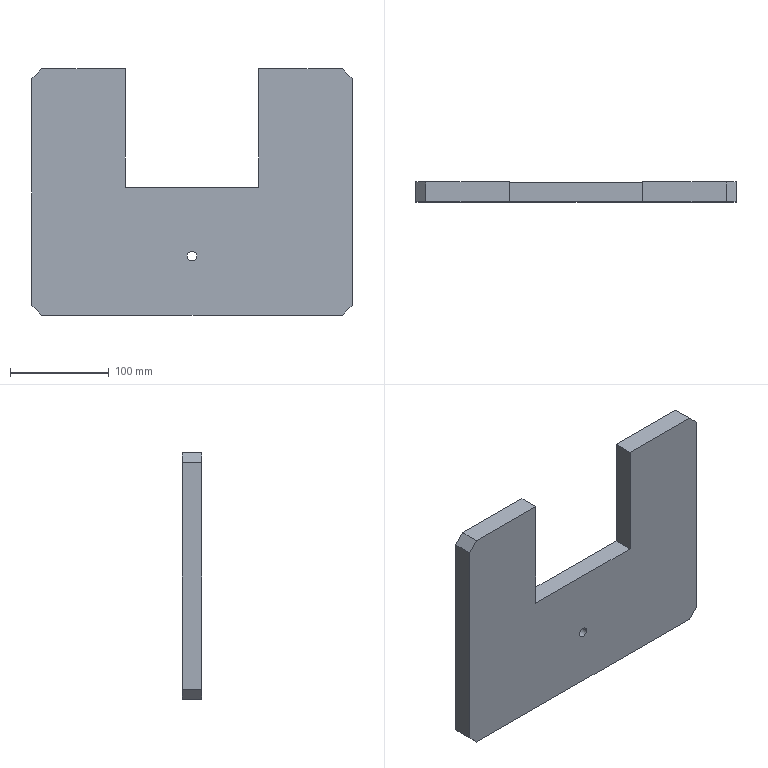Component | SolidWorks | RobotGripperBasePlateB-1 | 1 solid | 16 faces | box 325 x 20 x 250 mm | volume 1295429 mm3 | plane 14 | cylinder 2 | commonest cylinder face diameters 10 x2 | material Aviation Aluminum-7075
build123d program:
from build123d import *

# Parameters (mm, degrees)
SKETCH1_W           = 325
SKETCH1_H           = 250
BOSS_EXTRUDE1_DEPTH = 20
CHAMFER1_SIZE       = 10
SKETCH2_R           = 5
CUT_EXTRUDE1_DEPTH  = 206.988
CHAMFER2_SIZE       = 10
SKETCH3_W           = 135
SKETCH3_H           = 120
CUT_EXTRUDE2_DEPTH  = 206.988


with BuildPart() as part:
    # Sketch1 → Boss-Extrude1 (new body)
    with BuildSketch(Plane.XY):
        Rectangle(SKETCH1_W, SKETCH1_H)
    extrude(amount=BOSS_EXTRUDE1_DEPTH)

    # Chamfer1
    chamfer1_edges = [part.edges().sort_by_distance(p)[0] for p in [
        (-162.5, 125, 10),
        (162.5, 125, 10),
    ]]
    chamfer(chamfer1_edges, length=CHAMFER1_SIZE)

    # Sketch2 → Cut-Extrude1 (cut, through all)
    with BuildSketch(Plane.XY.offset(20)):
        with Locations((0, 65)):
            Circle(SKETCH2_R)
    extrude(amount=-CUT_EXTRUDE1_DEPTH, mode=Mode.SUBTRACT)

    # Chamfer2
    chamfer2_edges = [part.edges().sort_by_distance(p)[0] for p in [
        (162.5, -125, 10),
        (-162.5, -125, 10),
    ]]
    chamfer(chamfer2_edges, length=CHAMFER2_SIZE)

    # Sketch3 → Cut-Extrude2 (cut, through all)
    with BuildSketch(Plane(origin=(0, 0, 0), x_dir=(-1, 0, 0), z_dir=(0, 0, -1))):
        with Locations((0, -65)):
            Rectangle(SKETCH3_W, SKETCH3_H)
    extrude(amount=-CUT_EXTRUDE2_DEPTH, mode=Mode.SUBTRACT)


solid = part.part

# Placed as in the assembly
solid = solid.moved(Location((-47.37, -204.626, 352.215), (-90, 0, 0)))
STEP:
#1=COLOUR_RGB('',0.7922,0.8196,0.9333);
#2=FILL_AREA_STYLE_COLOUR('',#1);
#3=FILL_AREA_STYLE('',(#2));
#4=SURFACE_STYLE_FILL_AREA(#3);
#5=SURFACE_SIDE_STYLE('',(#4));
#6=SURFACE_STYLE_USAGE(.BOTH.,#5);
#7=PRESENTATION_STYLE_ASSIGNMENT((#6));
#8=CARTESIAN_POINT('',(-1.668,-7.269,11.308));
#9=VERTEX_POINT('',#8);
#10=CARTESIAN_POINT('',(-2.062,-7.269,11.308));
#11=VERTEX_POINT('',#10);
#12=CARTESIAN_POINT('',(-1.865,-7.269,11.308));
#13=DIRECTION('',(-0.,-1.,0.));
#14=DIRECTION('',(-1.,0.,0.));
#15=AXIS2_PLACEMENT_3D('',#12,#13,#14);
#16=CIRCLE('',#15,0.1969);
#17=EDGE_CURVE('',#9,#11,#16,.T.);
#18=ORIENTED_EDGE('',*,*,#17,.F.);
#19=CARTESIAN_POINT('',(-1.668,-8.056,11.308));
#20=VERTEX_POINT('',#19);
#21=CARTESIAN_POINT('',(-1.668,-7.269,11.308));
#22=DIRECTION('',(-0.,-1.,0.));
#23=VECTOR('',#22,39.37);
#24=LINE('',#21,#23);
#25=EDGE_CURVE('',#9,#20,#24,.T.);
#26=ORIENTED_EDGE('',*,*,#25,.T.);
#27=CARTESIAN_POINT('',(-2.062,-8.056,11.308));
#28=VERTEX_POINT('',#27);
#29=CARTESIAN_POINT('',(-1.865,-8.056,11.308));
#30=DIRECTION('',(-0.,-1.,0.));
#31=DIRECTION('',(-1.,0.,0.));
#32=AXIS2_PLACEMENT_3D('',#29,#30,#31);
#33=CIRCLE('',#32,0.1969);
#34=EDGE_CURVE('',#20,#28,#33,.T.);
#35=ORIENTED_EDGE('',*,*,#34,.T.);
#36=CARTESIAN_POINT('',(-2.062,-7.269,11.308));
#37=DIRECTION('',(-0.,-1.,0.));
#38=VECTOR('',#37,39.37);
#39=LINE('',#36,#38);
#40=EDGE_CURVE('',#11,#28,#39,.T.);
#41=ORIENTED_EDGE('',*,*,#40,.F.);
#42=EDGE_LOOP('',(#18,#26,#35,#41));
#43=FACE_OUTER_BOUND('',#42,.T.);
#44=CARTESIAN_POINT('',(-1.865,-7.269,11.308));
#45=DIRECTION('',(-0.,-1.,0.));
#46=DIRECTION('',(-1.,0.,0.));
#47=AXIS2_PLACEMENT_3D('',#44,#45,#46);
#48=CYLINDRICAL_SURFACE('',#47,0.1969);
#49=ADVANCED_FACE('',(#43),#48,.F.);
#50=CARTESIAN_POINT('',(-4.522,-8.056,18.788));
#51=VERTEX_POINT('',#50);
#52=CARTESIAN_POINT('',(-7.869,-8.056,18.788));
#53=VERTEX_POINT('',#52);
#54=CARTESIAN_POINT('',(-8.263,-8.056,18.788));
#55=DIRECTION('',(-1.,0.,0.));
#56=VECTOR('',#55,39.37);
#57=LINE('',#54,#56);
#58=EDGE_CURVE('',#51,#53,#57,.T.);
#59=ORIENTED_EDGE('',*,*,#58,.F.);
#60=CARTESIAN_POINT('',(-4.522,-7.269,18.788));
#61=VERTEX_POINT('',#60);
#62=CARTESIAN_POINT('',(-4.522,-8.056,18.788));
#63=DIRECTION('',(0.,1.,0.));
#64=VECTOR('',#63,39.37);
#65=LINE('',#62,#64);
#66=EDGE_CURVE('',#51,#61,#65,.T.);
#67=ORIENTED_EDGE('',*,*,#66,.T.);
#68=CARTESIAN_POINT('',(-7.869,-7.269,18.788));
#69=VERTEX_POINT('',#68);
#70=CARTESIAN_POINT('',(-8.263,-7.269,18.788));
#71=DIRECTION('',(-1.,0.,0.));
#72=VECTOR('',#71,39.37);
#73=LINE('',#70,#72);
#74=EDGE_CURVE('',#61,#69,#73,.T.);
#75=ORIENTED_EDGE('',*,*,#74,.T.);
#76=CARTESIAN_POINT('',(-7.869,-8.056,18.788));
#77=DIRECTION('',(-0.,-1.,0.));
#78=VECTOR('',#77,39.37);
#79=LINE('',#76,#78);
#80=EDGE_CURVE('',#69,#53,#79,.T.);
#81=ORIENTED_EDGE('',*,*,#80,.T.);
#82=EDGE_LOOP('',(#59,#67,#75,#81));
#83=FACE_OUTER_BOUND('',#82,.T.);
#84=CARTESIAN_POINT('',(-8.263,-8.056,18.788));
#85=DIRECTION('',(-0.,0.,-1.));
#86=DIRECTION('',(1.,-0.,-0.));
#87=AXIS2_PLACEMENT_3D('',#84,#85,#86);
#88=PLANE('',#87);
#89=ADVANCED_FACE('',(#83),#88,.F.);
#90=CARTESIAN_POINT('',(4.533,-7.269,9.339));
#91=VERTEX_POINT('',#90);
#92=CARTESIAN_POINT('',(4.533,-7.269,18.394));
#93=VERTEX_POINT('',#92);
#94=CARTESIAN_POINT('',(4.533,-7.269,18.788));
#95=DIRECTION('',(0.,-0.,1.));
#96=VECTOR('',#95,39.37);
#97=LINE('',#94,#96);
#98=EDGE_CURVE('',#91,#93,#97,.T.);
#99=ORIENTED_EDGE('',*,*,#98,.T.);
#100=CARTESIAN_POINT('',(4.533,-8.056,18.394));
#101=VERTEX_POINT('',#100);
#102=CARTESIAN_POINT('',(4.533,-8.056,18.394));
#103=DIRECTION('',(-0.,-1.,0.));
#104=VECTOR('',#103,39.37);
#105=LINE('',#102,#104);
#106=EDGE_CURVE('',#93,#101,#105,.T.);
#107=ORIENTED_EDGE('',*,*,#106,.T.);
#108=CARTESIAN_POINT('',(4.533,-8.056,9.339));
#109=VERTEX_POINT('',#108);
#110=CARTESIAN_POINT('',(4.533,-8.056,18.788));
#111=DIRECTION('',(0.,-0.,1.));
#112=VECTOR('',#111,39.37);
#113=LINE('',#110,#112);
#114=EDGE_CURVE('',#109,#101,#113,.T.);
#115=ORIENTED_EDGE('',*,*,#114,.F.);
#116=CARTESIAN_POINT('',(4.533,-8.056,9.339));
#117=DIRECTION('',(0.,1.,0.));
#118=VECTOR('',#117,39.37);
#119=LINE('',#116,#118);
#120=EDGE_CURVE('',#109,#91,#119,.T.);
#121=ORIENTED_EDGE('',*,*,#120,.T.);
#122=EDGE_LOOP('',(#99,#107,#115,#121));
#123=FACE_OUTER_BOUND('',#122,.T.);
#124=CARTESIAN_POINT('',(4.533,-8.056,18.788));
#125=DIRECTION('',(-1.,0.,0.));
#126=DIRECTION('',(0.,1.,0.));
#127=AXIS2_PLACEMENT_3D('',#124,#125,#126);
#128=PLANE('',#127);
#129=ADVANCED_FACE('',(#123),#128,.F.);
#130=CARTESIAN_POINT('',(4.139,-7.269,18.788));
#131=VERTEX_POINT('',#130);
#132=CARTESIAN_POINT('',(0.7925,-7.269,18.788));
#133=VERTEX_POINT('',#132);
#134=CARTESIAN_POINT('',(-8.263,-7.269,18.788));
#135=DIRECTION('',(-1.,0.,0.));
#136=VECTOR('',#135,39.37);
#137=LINE('',#134,#136);
#138=EDGE_CURVE('',#131,#133,#137,.T.);
#139=ORIENTED_EDGE('',*,*,#138,.T.);
#140=CARTESIAN_POINT('',(0.7925,-8.056,18.788));
#141=VERTEX_POINT('',#140);
#142=CARTESIAN_POINT('',(0.7925,-8.056,18.788));
#143=DIRECTION('',(0.,1.,0.));
#144=VECTOR('',#143,39.37);
#145=LINE('',#142,#144);
#146=EDGE_CURVE('',#141,#133,#145,.T.);
#147=ORIENTED_EDGE('',*,*,#146,.F.);
#148=CARTESIAN_POINT('',(4.139,-8.056,18.788));
#149=VERTEX_POINT('',#148);
#150=CARTESIAN_POINT('',(-8.263,-8.056,18.788));
#151=DIRECTION('',(-1.,0.,0.));
#152=VECTOR('',#151,39.37);
#153=LINE('',#150,#152);
#154=EDGE_CURVE('',#149,#141,#153,.T.);
#155=ORIENTED_EDGE('',*,*,#154,.F.);
#156=CARTESIAN_POINT('',(4.139,-8.056,18.788));
#157=DIRECTION('',(0.,1.,0.));
#158=VECTOR('',#157,39.37);
#159=LINE('',#156,#158);
#160=EDGE_CURVE('',#149,#131,#159,.T.);
#161=ORIENTED_EDGE('',*,*,#160,.T.);
#162=EDGE_LOOP('',(#139,#147,#155,#161));
#163=FACE_OUTER_BOUND('',#162,.T.);
#164=CARTESIAN_POINT('',(-8.263,-8.056,18.788));
#165=DIRECTION('',(-0.,0.,-1.));
#166=DIRECTION('',(1.,-0.,-0.));
#167=AXIS2_PLACEMENT_3D('',#164,#165,#166);
#168=PLANE('',#167);
#169=ADVANCED_FACE('',(#163),#168,.F.);
#170=CARTESIAN_POINT('',(-8.263,-8.056,18.394));
#171=VERTEX_POINT('',#170);
#172=CARTESIAN_POINT('',(-8.263,-8.056,9.339));
#173=VERTEX_POINT('',#172);
#174=CARTESIAN_POINT('',(-8.263,-8.056,18.788));
#175=DIRECTION('',(-0.,0.,-1.));
#176=VECTOR('',#175,39.37);
#177=LINE('',#174,#176);
#178=EDGE_CURVE('',#171,#173,#177,.T.);
#179=ORIENTED_EDGE('',*,*,#178,.F.);
#180=CARTESIAN_POINT('',(-8.263,-7.269,18.394));
#181=VERTEX_POINT('',#180);
#182=CARTESIAN_POINT('',(-8.263,-8.056,18.394));
#183=DIRECTION('',(0.,1.,0.));
#184=VECTOR('',#183,39.37);
#185=LINE('',#182,#184);
#186=EDGE_CURVE('',#171,#181,#185,.T.);
#187=ORIENTED_EDGE('',*,*,#186,.T.);
#188=CARTESIAN_POINT('',(-8.263,-7.269,9.339));
#189=VERTEX_POINT('',#188);
#190=CARTESIAN_POINT('',(-8.263,-7.269,18.788));
#191=DIRECTION('',(-0.,0.,-1.));
#192=VECTOR('',#191,39.37);
#193=LINE('',#190,#192);
#194=EDGE_CURVE('',#181,#189,#193,.T.);
#195=ORIENTED_EDGE('',*,*,#194,.T.);
#196=CARTESIAN_POINT('',(-8.263,-8.056,9.339));
#197=DIRECTION('',(-0.,-1.,0.));
#198=VECTOR('',#197,39.37);
#199=LINE('',#196,#198);
#200=EDGE_CURVE('',#189,#173,#199,.T.);
#201=ORIENTED_EDGE('',*,*,#200,.T.);
#202=EDGE_LOOP('',(#179,#187,#195,#201));
#203=FACE_OUTER_BOUND('',#202,.T.);
#204=CARTESIAN_POINT('',(-8.263,-8.056,18.788));
#205=DIRECTION('',(1.,-0.,-0.));
#206=DIRECTION('',(-0.,-1.,0.));
#207=AXIS2_PLACEMENT_3D('',#204,#205,#206);
#208=PLANE('',#207);
#209=ADVANCED_FACE('',(#203),#208,.F.);
#210=CARTESIAN_POINT('',(-7.869,-8.056,8.945));
#211=VERTEX_POINT('',#210);
#212=CARTESIAN_POINT('',(4.139,-8.056,8.945));
#213=VERTEX_POINT('',#212);
#214=CARTESIAN_POINT('',(-8.263,-8.056,8.945));
#215=DIRECTION('',(1.,-0.,-0.));
#216=VECTOR('',#215,39.37);
#217=LINE('',#214,#216);
#218=EDGE_CURVE('',#211,#213,#217,.T.);
#219=ORIENTED_EDGE('',*,*,#218,.F.);
#220=CARTESIAN_POINT('',(-7.869,-7.269,8.945));
#221=VERTEX_POINT('',#220);
#222=CARTESIAN_POINT('',(-7.869,-8.056,8.945));
#223=DIRECTION('',(0.,1.,0.));
#224=VECTOR('',#223,39.37);
#225=LINE('',#222,#224);
#226=EDGE_CURVE('',#211,#221,#225,.T.);
#227=ORIENTED_EDGE('',*,*,#226,.T.);
#228=CARTESIAN_POINT('',(4.139,-7.269,8.945));
#229=VERTEX_POINT('',#228);
#230=CARTESIAN_POINT('',(-8.263,-7.269,8.945));
#231=DIRECTION('',(1.,-0.,-0.));
#232=VECTOR('',#231,39.37);
#233=LINE('',#230,#232);
#234=EDGE_CURVE('',#221,#229,#233,.T.);
#235=ORIENTED_EDGE('',*,*,#234,.T.);
#236=CARTESIAN_POINT('',(4.139,-8.056,8.945));
#237=DIRECTION('',(-0.,-1.,0.));
#238=VECTOR('',#237,39.37);
#239=LINE('',#236,#238);
#240=EDGE_CURVE('',#229,#213,#239,.T.);
#241=ORIENTED_EDGE('',*,*,#240,.T.);
#242=EDGE_LOOP('',(#219,#227,#235,#241));
#243=FACE_OUTER_BOUND('',#242,.T.);
#244=CARTESIAN_POINT('',(-8.263,-8.056,8.945));
#245=DIRECTION('',(0.,-0.,1.));
#246=DIRECTION('',(-1.,0.,0.));
#247=AXIS2_PLACEMENT_3D('',#244,#245,#246);
#248=PLANE('',#247);
#249=ADVANCED_FACE('',(#243),#248,.F.);
#250=CARTESIAN_POINT('',(-4.522,-8.056,14.064));
#251=VERTEX_POINT('',#250);
#252=CARTESIAN_POINT('',(-4.522,-8.056,14.064));
#253=DIRECTION('',(0.,-0.,1.));
#254=VECTOR('',#253,39.37);
#255=LINE('',#252,#254);
#256=EDGE_CURVE('',#251,#51,#255,.T.);
#257=ORIENTED_EDGE('',*,*,#256,.T.);
#258=ORIENTED_EDGE('',*,*,#58,.T.);
#259=CARTESIAN_POINT('',(-7.328,-8.056,19.329));
#260=DIRECTION('',(-0.7071,0.,-0.7071));
#261=VECTOR('',#260,39.37);
#262=LINE('',#259,#261);
#263=EDGE_CURVE('',#53,#171,#262,.T.);
#264=ORIENTED_EDGE('',*,*,#263,.T.);
#265=ORIENTED_EDGE('',*,*,#178,.T.);
#266=CARTESIAN_POINT('',(-7.328,-8.056,8.404));
#267=DIRECTION('',(0.7071,-0.,-0.7071));
#268=VECTOR('',#267,39.37);
#269=LINE('',#266,#268);
#270=EDGE_CURVE('',#173,#211,#269,.T.);
#271=ORIENTED_EDGE('',*,*,#270,.T.);
#272=ORIENTED_EDGE('',*,*,#218,.T.);
#273=CARTESIAN_POINT('',(3.598,-8.056,8.404));
#274=DIRECTION('',(0.7071,-0.,0.7071));
#275=VECTOR('',#274,39.37);
#276=LINE('',#273,#275);
#277=EDGE_CURVE('',#213,#109,#276,.T.);
#278=ORIENTED_EDGE('',*,*,#277,.T.);
#279=ORIENTED_EDGE('',*,*,#114,.T.);
#280=CARTESIAN_POINT('',(3.598,-8.056,19.329));
#281=DIRECTION('',(-0.7071,0.,0.7071));
#282=VECTOR('',#281,39.37);
#283=LINE('',#280,#282);
#284=EDGE_CURVE('',#101,#149,#283,.T.);
#285=ORIENTED_EDGE('',*,*,#284,.T.);
#286=ORIENTED_EDGE('',*,*,#154,.T.);
#287=CARTESIAN_POINT('',(0.7925,-8.056,14.064));
#288=VERTEX_POINT('',#287);
#289=CARTESIAN_POINT('',(0.7925,-8.056,14.064));
#290=DIRECTION('',(-0.,0.,-1.));
#291=VECTOR('',#290,39.37);
#292=LINE('',#289,#291);
#293=EDGE_CURVE('',#141,#288,#292,.T.);
#294=ORIENTED_EDGE('',*,*,#293,.T.);
#295=CARTESIAN_POINT('',(0.7925,-8.056,14.064));
#296=DIRECTION('',(-1.,0.,0.));
#297=VECTOR('',#296,39.37);
#298=LINE('',#295,#297);
#299=EDGE_CURVE('',#288,#251,#298,.T.);
#300=ORIENTED_EDGE('',*,*,#299,.T.);
#301=EDGE_LOOP('',(#257,#258,#264,#265,#271,#272,#278,#279,#285,#286,#294,#300));
#302=FACE_OUTER_BOUND('',#301,.T.);
#303=CARTESIAN_POINT('',(-1.865,-8.056,11.308));
#304=DIRECTION('',(-0.,-1.,0.));
#305=DIRECTION('',(-1.,0.,0.));
#306=AXIS2_PLACEMENT_3D('',#303,#304,#305);
#307=CIRCLE('',#306,0.1969);
#308=EDGE_CURVE('',#28,#20,#307,.T.);
#309=ORIENTED_EDGE('',*,*,#308,.F.);
#310=ORIENTED_EDGE('',*,*,#34,.F.);
#311=EDGE_LOOP('',(#309,#310));
#312=FACE_BOUND('',#311,.T.);
#313=CARTESIAN_POINT('',(-1.865,-8.056,13.867));
#314=DIRECTION('',(-0.,-1.,0.));
#315=DIRECTION('',(-1.,0.,0.));
#316=AXIS2_PLACEMENT_3D('',#313,#314,#315);
#317=PLANE('',#316);
#318=ADVANCED_FACE('',(#302,#312),#317,.T.);
#319=CARTESIAN_POINT('',(-1.865,-7.269,11.308));
#320=DIRECTION('',(-0.,-1.,0.));
#321=DIRECTION('',(-1.,0.,0.));
#322=AXIS2_PLACEMENT_3D('',#319,#320,#321);
#323=CIRCLE('',#322,0.1969);
#324=EDGE_CURVE('',#11,#9,#323,.T.);
#325=ORIENTED_EDGE('',*,*,#324,.T.);
#326=ORIENTED_EDGE('',*,*,#17,.T.);
#327=EDGE_LOOP('',(#325,#326));
#328=FACE_BOUND('',#327,.T.);
#329=ORIENTED_EDGE('',*,*,#74,.F.);
#330=CARTESIAN_POINT('',(-4.522,-7.269,14.064));
#331=VERTEX_POINT('',#330);
#332=CARTESIAN_POINT('',(-4.522,-7.269,14.064));
#333=DIRECTION('',(0.,-0.,1.));
#334=VECTOR('',#333,39.37);
#335=LINE('',#332,#334);
#336=EDGE_CURVE('',#331,#61,#335,.T.);
#337=ORIENTED_EDGE('',*,*,#336,.F.);
#338=CARTESIAN_POINT('',(0.7925,-7.269,14.064));
#339=VERTEX_POINT('',#338);
#340=CARTESIAN_POINT('',(0.7925,-7.269,14.064));
#341=DIRECTION('',(-1.,0.,0.));
#342=VECTOR('',#341,39.37);
#343=LINE('',#340,#342);
#344=EDGE_CURVE('',#339,#331,#343,.T.);
#345=ORIENTED_EDGE('',*,*,#344,.F.);
#346=CARTESIAN_POINT('',(0.7925,-7.269,14.064));
#347=DIRECTION('',(-0.,0.,-1.));
#348=VECTOR('',#347,39.37);
#349=LINE('',#346,#348);
#350=EDGE_CURVE('',#133,#339,#349,.T.);
#351=ORIENTED_EDGE('',*,*,#350,.F.);
#352=ORIENTED_EDGE('',*,*,#138,.F.);
#353=CARTESIAN_POINT('',(4.139,-7.269,18.788));
#354=DIRECTION('',(0.7071,-0.,-0.7071));
#355=VECTOR('',#354,39.37);
#356=LINE('',#353,#355);
#357=EDGE_CURVE('',#131,#93,#356,.T.);
#358=ORIENTED_EDGE('',*,*,#357,.T.);
#359=ORIENTED_EDGE('',*,*,#98,.F.);
#360=CARTESIAN_POINT('',(4.533,-7.269,9.339));
#361=DIRECTION('',(-0.7071,0.,-0.7071));
#362=VECTOR('',#361,39.37);
#363=LINE('',#360,#362);
#364=EDGE_CURVE('',#91,#229,#363,.T.);
#365=ORIENTED_EDGE('',*,*,#364,.T.);
#366=ORIENTED_EDGE('',*,*,#234,.F.);
#367=CARTESIAN_POINT('',(-7.869,-7.269,8.945));
#368=DIRECTION('',(-0.7071,0.,0.7071));
#369=VECTOR('',#368,39.37);
#370=LINE('',#367,#369);
#371=EDGE_CURVE('',#221,#189,#370,.T.);
#372=ORIENTED_EDGE('',*,*,#371,.T.);
#373=ORIENTED_EDGE('',*,*,#194,.F.);
#374=CARTESIAN_POINT('',(-8.263,-7.269,18.394));
#375=DIRECTION('',(0.7071,-0.,0.7071));
#376=VECTOR('',#375,39.37);
#377=LINE('',#374,#376);
#378=EDGE_CURVE('',#181,#69,#377,.T.);
#379=ORIENTED_EDGE('',*,*,#378,.T.);
#380=EDGE_LOOP('',(#329,#337,#345,#351,#352,#358,#359,#365,#366,#372,#373,#379));
#381=FACE_OUTER_BOUND('',#380,.T.);
#382=CARTESIAN_POINT('',(-1.865,-7.269,13.867));
#383=DIRECTION('',(-0.,-1.,0.));
#384=DIRECTION('',(-1.,0.,0.));
#385=AXIS2_PLACEMENT_3D('',#382,#383,#384);
#386=PLANE('',#385);
#387=ADVANCED_FACE('',(#328,#381),#386,.F.);
#388=ORIENTED_EDGE('',*,*,#270,.F.);
#389=ORIENTED_EDGE('',*,*,#200,.F.);
#390=ORIENTED_EDGE('',*,*,#371,.F.);
#391=ORIENTED_EDGE('',*,*,#226,.F.);
#392=EDGE_LOOP('',(#388,#389,#390,#391));
#393=FACE_OUTER_BOUND('',#392,.T.);
#394=CARTESIAN_POINT('',(-7.869,-8.056,8.945));
#395=DIRECTION('',(0.7071,-0.,0.7071));
#396=DIRECTION('',(0.,1.,0.));
#397=AXIS2_PLACEMENT_3D('',#394,#395,#396);
#398=PLANE('',#397);
#399=ADVANCED_FACE('',(#393),#398,.F.);
#400=ORIENTED_EDGE('',*,*,#277,.F.);
#401=ORIENTED_EDGE('',*,*,#240,.F.);
#402=ORIENTED_EDGE('',*,*,#364,.F.);
#403=ORIENTED_EDGE('',*,*,#120,.F.);
#404=EDGE_LOOP('',(#400,#401,#402,#403));
#405=FACE_OUTER_BOUND('',#404,.T.);
#406=CARTESIAN_POINT('',(4.533,-8.056,9.339));
#407=DIRECTION('',(-0.7071,0.,0.7071));
#408=DIRECTION('',(0.,1.,0.));
#409=AXIS2_PLACEMENT_3D('',#406,#407,#408);
#410=PLANE('',#409);
#411=ADVANCED_FACE('',(#405),#410,.F.);
#412=ORIENTED_EDGE('',*,*,#25,.F.);
#413=ORIENTED_EDGE('',*,*,#324,.F.);
#414=ORIENTED_EDGE('',*,*,#40,.T.);
#415=ORIENTED_EDGE('',*,*,#308,.T.);
#416=EDGE_LOOP('',(#412,#413,#414,#415));
#417=FACE_OUTER_BOUND('',#416,.T.);
#418=CARTESIAN_POINT('',(-1.865,-7.269,11.308));
#419=DIRECTION('',(-0.,-1.,0.));
#420=DIRECTION('',(-1.,0.,0.));
#421=AXIS2_PLACEMENT_3D('',#418,#419,#420);
#422=CYLINDRICAL_SURFACE('',#421,0.1969);
#423=ADVANCED_FACE('',(#417),#422,.F.);
#424=ORIENTED_EDGE('',*,*,#263,.F.);
#425=ORIENTED_EDGE('',*,*,#80,.F.);
#426=ORIENTED_EDGE('',*,*,#378,.F.);
#427=ORIENTED_EDGE('',*,*,#186,.F.);
#428=EDGE_LOOP('',(#424,#425,#426,#427));
#429=FACE_OUTER_BOUND('',#428,.T.);
#430=CARTESIAN_POINT('',(-8.263,-8.056,18.394));
#431=DIRECTION('',(0.7071,-0.,-0.7071));
#432=DIRECTION('',(0.,1.,0.));
#433=AXIS2_PLACEMENT_3D('',#430,#431,#432);
#434=PLANE('',#433);
#435=ADVANCED_FACE('',(#429),#434,.F.);
#436=ORIENTED_EDGE('',*,*,#284,.F.);
#437=ORIENTED_EDGE('',*,*,#106,.F.);
#438=ORIENTED_EDGE('',*,*,#357,.F.);
#439=ORIENTED_EDGE('',*,*,#160,.F.);
#440=EDGE_LOOP('',(#436,#437,#438,#439));
#441=FACE_OUTER_BOUND('',#440,.T.);
#442=CARTESIAN_POINT('',(4.139,-8.056,18.788));
#443=DIRECTION('',(-0.7071,0.,-0.7071));
#444=DIRECTION('',(0.,1.,0.));
#445=AXIS2_PLACEMENT_3D('',#442,#443,#444);
#446=PLANE('',#445);
#447=ADVANCED_FACE('',(#441),#446,.F.);
#448=ORIENTED_EDGE('',*,*,#336,.T.);
#449=ORIENTED_EDGE('',*,*,#66,.F.);
#450=ORIENTED_EDGE('',*,*,#256,.F.);
#451=CARTESIAN_POINT('',(-4.522,-8.056,14.064));
#452=DIRECTION('',(0.,1.,0.));
#453=VECTOR('',#452,39.37);
#454=LINE('',#451,#453);
#455=EDGE_CURVE('',#251,#331,#454,.T.);
#456=ORIENTED_EDGE('',*,*,#455,.T.);
#457=EDGE_LOOP('',(#448,#449,#450,#456));
#458=FACE_OUTER_BOUND('',#457,.T.);
#459=CARTESIAN_POINT('',(-4.522,-8.056,14.064));
#460=DIRECTION('',(-1.,0.,0.));
#461=DIRECTION('',(-0.,0.,-1.));
#462=AXIS2_PLACEMENT_3D('',#459,#460,#461);
#463=PLANE('',#462);
#464=ADVANCED_FACE('',(#458),#463,.F.);
#465=ORIENTED_EDGE('',*,*,#344,.T.);
#466=ORIENTED_EDGE('',*,*,#455,.F.);
#467=ORIENTED_EDGE('',*,*,#299,.F.);
#468=CARTESIAN_POINT('',(0.7925,-8.056,14.064));
#469=DIRECTION('',(0.,1.,0.));
#470=VECTOR('',#469,39.37);
#471=LINE('',#468,#470);
#472=EDGE_CURVE('',#288,#339,#471,.T.);
#473=ORIENTED_EDGE('',*,*,#472,.T.);
#474=EDGE_LOOP('',(#465,#466,#467,#473));
#475=FACE_OUTER_BOUND('',#474,.T.);
#476=CARTESIAN_POINT('',(0.7925,-8.056,14.064));
#477=DIRECTION('',(-0.,0.,-1.));
#478=DIRECTION('',(1.,-0.,-0.));
#479=AXIS2_PLACEMENT_3D('',#476,#477,#478);
#480=PLANE('',#479);
#481=ADVANCED_FACE('',(#475),#480,.F.);
#482=ORIENTED_EDGE('',*,*,#350,.T.);
#483=ORIENTED_EDGE('',*,*,#472,.F.);
#484=ORIENTED_EDGE('',*,*,#293,.F.);
#485=ORIENTED_EDGE('',*,*,#146,.T.);
#486=EDGE_LOOP('',(#482,#483,#484,#485));
#487=FACE_OUTER_BOUND('',#486,.T.);
#488=CARTESIAN_POINT('',(0.7925,-8.056,14.064));
#489=DIRECTION('',(1.,-0.,-0.));
#490=DIRECTION('',(0.,-0.,1.));
#491=AXIS2_PLACEMENT_3D('',#488,#489,#490);
#492=PLANE('',#491);
#493=ADVANCED_FACE('',(#487),#492,.F.);
#494=CLOSED_SHELL('',(#49,#89,#129,#169,#209,#249,#318,#387,#399,#411,#423,#435,#447,#464,#481,#493));
#495=MANIFOLD_SOLID_BREP('',#494);
#496=STYLED_ITEM('',(#7),#495);
#497=(LENGTH_UNIT()NAMED_UNIT(*)SI_UNIT($,.METRE.));
#498=LENGTH_MEASURE_WITH_UNIT(LENGTH_MEASURE(0.0254),#497);
#499=DIMENSIONAL_EXPONENTS(1.,0.,0.,0.,0.,0.,0.);
#500=(CONVERSION_BASED_UNIT('',#498)LENGTH_UNIT()NAMED_UNIT(#499));
#501=UNCERTAINTY_MEASURE_WITH_UNIT(LENGTH_MEASURE(0.00001),#500,'','');
#502=(NAMED_UNIT(*)PLANE_ANGLE_UNIT()SI_UNIT($,.RADIAN.));
#503=(NAMED_UNIT(*)SI_UNIT($,.STERADIAN.)SOLID_ANGLE_UNIT());
#504=(GEOMETRIC_REPRESENTATION_CONTEXT(3)GLOBAL_UNCERTAINTY_ASSIGNED_CONTEXT((#501))GLOBAL_UNIT_ASSIGNED_CONTEXT((#500,#502,#503))REPRESENTATION_CONTEXT('',''));
#505=MECHANICAL_DESIGN_GEOMETRIC_PRESENTATION_REPRESENTATION('',(#496),#504);
#506=CARTESIAN_POINT('',(0.,0.,0.));
#507=DIRECTION('',(0.,0.,1.));
#508=DIRECTION('',(1.,0.,0.));
#509=AXIS2_PLACEMENT_3D('',#506,#507,#508);
#510=(LENGTH_UNIT()NAMED_UNIT(*)SI_UNIT($,.METRE.));
#511=LENGTH_MEASURE_WITH_UNIT(LENGTH_MEASURE(0.0254),#510);
#512=DIMENSIONAL_EXPONENTS(1.,0.,0.,0.,0.,0.,0.);
#513=(CONVERSION_BASED_UNIT('',#511)LENGTH_UNIT()NAMED_UNIT(#512));
#514=UNCERTAINTY_MEASURE_WITH_UNIT(LENGTH_MEASURE(0.00001),#513,'','');
#515=(NAMED_UNIT(*)PLANE_ANGLE_UNIT()SI_UNIT($,.RADIAN.));
#516=(NAMED_UNIT(*)SI_UNIT($,.STERADIAN.)SOLID_ANGLE_UNIT());
#517=(GEOMETRIC_REPRESENTATION_CONTEXT(3)GLOBAL_UNCERTAINTY_ASSIGNED_CONTEXT((#514))GLOBAL_UNIT_ASSIGNED_CONTEXT((#513,#515,#516))REPRESENTATION_CONTEXT('',''));
#518=ADVANCED_BREP_SHAPE_REPRESENTATION('',(#495,#509),#517);
#519=PRESENTATION_LAYER_ASSIGNMENT('','',(#496));